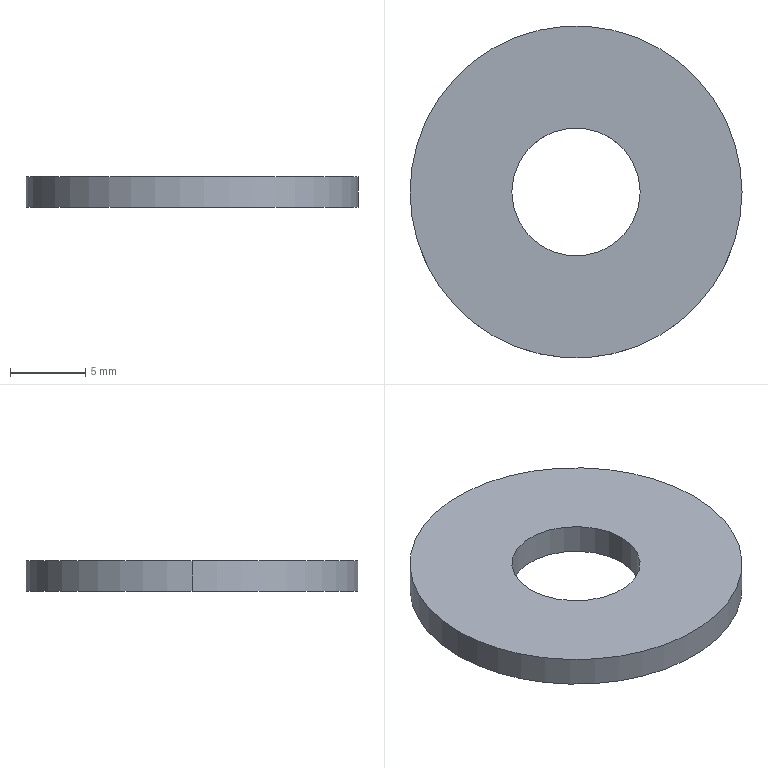Component | SolidWorks | 8mmLargeWasher-1 | 1 solid | 6 faces | box 22 x 22 x 2 mm | volume 647 mm3 | cylinder 4 | plane 2 | commonest cylinder face diameters 8.5 x2 22 x2
build123d program:
from build123d import *

# Parameters (mm, degrees)
SKETCH1_R           = 11
SKETCH1_R_2         = 4.25
BOSS_EXTRUDE1_DEPTH = 2


with BuildPart() as part:
    # Sketch1 → Boss-Extrude1 (new body)
    with BuildSketch(Plane.XY):
        with Locations((-70, -20)):
            Circle(SKETCH1_R)
        with Locations((-70, -20)):
            Circle(SKETCH1_R_2, mode=Mode.SUBTRACT)
    extrude(amount=BOSS_EXTRUDE1_DEPTH)


solid = part.part

# Placed as in the assembly
solid = solid.moved(Location((-426.612, -103.873, 2355.4), (0, 0, 0)))
STEP:
#1=COLOUR_RGB('',0.7922,0.8196,0.9333);
#2=FILL_AREA_STYLE_COLOUR('',#1);
#3=FILL_AREA_STYLE('',(#2));
#4=SURFACE_STYLE_FILL_AREA(#3);
#5=SURFACE_SIDE_STYLE('',(#4));
#6=SURFACE_STYLE_USAGE(.BOTH.,#5);
#7=PRESENTATION_STYLE_ASSIGNMENT((#6));
#8=CARTESIAN_POINT('',(-19.719,-4.877,92.732));
#9=VERTEX_POINT('',#8);
#10=CARTESIAN_POINT('',(-19.384,-4.877,92.732));
#11=VERTEX_POINT('',#10);
#12=CARTESIAN_POINT('',(-19.552,-4.877,92.732));
#13=DIRECTION('',(0.,0.,-1.));
#14=DIRECTION('',(1.,0.,0.));
#15=AXIS2_PLACEMENT_3D('',#12,#13,#14);
#16=CIRCLE('',#15,0.1673);
#17=EDGE_CURVE('',#9,#11,#16,.T.);
#18=ORIENTED_EDGE('',*,*,#17,.T.);
#19=CARTESIAN_POINT('',(-19.384,-4.877,92.811));
#20=VERTEX_POINT('',#19);
#21=CARTESIAN_POINT('',(-19.384,-4.877,92.732));
#22=DIRECTION('',(0.,-0.,1.));
#23=VECTOR('',#22,39.37);
#24=LINE('',#21,#23);
#25=EDGE_CURVE('',#11,#20,#24,.T.);
#26=ORIENTED_EDGE('',*,*,#25,.T.);
#27=CARTESIAN_POINT('',(-19.719,-4.877,92.811));
#28=VERTEX_POINT('',#27);
#29=CARTESIAN_POINT('',(-19.552,-4.877,92.811));
#30=DIRECTION('',(0.,0.,-1.));
#31=DIRECTION('',(1.,0.,0.));
#32=AXIS2_PLACEMENT_3D('',#29,#30,#31);
#33=CIRCLE('',#32,0.1673);
#34=EDGE_CURVE('',#28,#20,#33,.T.);
#35=ORIENTED_EDGE('',*,*,#34,.F.);
#36=CARTESIAN_POINT('',(-19.719,-4.877,92.732));
#37=DIRECTION('',(0.,-0.,1.));
#38=VECTOR('',#37,39.37);
#39=LINE('',#36,#38);
#40=EDGE_CURVE('',#9,#28,#39,.T.);
#41=ORIENTED_EDGE('',*,*,#40,.F.);
#42=EDGE_LOOP('',(#18,#26,#35,#41));
#43=FACE_OUTER_BOUND('',#42,.T.);
#44=CARTESIAN_POINT('',(-19.552,-4.877,92.732));
#45=DIRECTION('',(0.,-0.,1.));
#46=DIRECTION('',(-1.,0.,0.));
#47=AXIS2_PLACEMENT_3D('',#44,#45,#46);
#48=CYLINDRICAL_SURFACE('',#47,0.1673);
#49=ADVANCED_FACE('',(#43),#48,.F.);
#50=CARTESIAN_POINT('',(-19.119,-4.877,92.732));
#51=VERTEX_POINT('',#50);
#52=CARTESIAN_POINT('',(-19.985,-4.877,92.732));
#53=VERTEX_POINT('',#52);
#54=CARTESIAN_POINT('',(-19.552,-4.877,92.732));
#55=DIRECTION('',(0.,0.,-1.));
#56=DIRECTION('',(1.,0.,0.));
#57=AXIS2_PLACEMENT_3D('',#54,#55,#56);
#58=CIRCLE('',#57,0.4331);
#59=EDGE_CURVE('',#51,#53,#58,.T.);
#60=ORIENTED_EDGE('',*,*,#59,.F.);
#61=CARTESIAN_POINT('',(-19.119,-4.877,92.811));
#62=VERTEX_POINT('',#61);
#63=CARTESIAN_POINT('',(-19.119,-4.877,92.732));
#64=DIRECTION('',(0.,-0.,1.));
#65=VECTOR('',#64,39.37);
#66=LINE('',#63,#65);
#67=EDGE_CURVE('',#51,#62,#66,.T.);
#68=ORIENTED_EDGE('',*,*,#67,.T.);
#69=CARTESIAN_POINT('',(-19.985,-4.877,92.811));
#70=VERTEX_POINT('',#69);
#71=CARTESIAN_POINT('',(-19.552,-4.877,92.811));
#72=DIRECTION('',(0.,0.,-1.));
#73=DIRECTION('',(1.,0.,0.));
#74=AXIS2_PLACEMENT_3D('',#71,#72,#73);
#75=CIRCLE('',#74,0.4331);
#76=EDGE_CURVE('',#62,#70,#75,.T.);
#77=ORIENTED_EDGE('',*,*,#76,.T.);
#78=CARTESIAN_POINT('',(-19.985,-4.877,92.732));
#79=DIRECTION('',(0.,-0.,1.));
#80=VECTOR('',#79,39.37);
#81=LINE('',#78,#80);
#82=EDGE_CURVE('',#53,#70,#81,.T.);
#83=ORIENTED_EDGE('',*,*,#82,.F.);
#84=EDGE_LOOP('',(#60,#68,#77,#83));
#85=FACE_OUTER_BOUND('',#84,.T.);
#86=CARTESIAN_POINT('',(-19.552,-4.877,92.732));
#87=DIRECTION('',(0.,-0.,1.));
#88=DIRECTION('',(-1.,0.,0.));
#89=AXIS2_PLACEMENT_3D('',#86,#87,#88);
#90=CYLINDRICAL_SURFACE('',#89,0.4331);
#91=ADVANCED_FACE('',(#85),#90,.T.);
#92=CARTESIAN_POINT('',(-19.552,-4.877,92.732));
#93=DIRECTION('',(0.,0.,-1.));
#94=DIRECTION('',(1.,0.,0.));
#95=AXIS2_PLACEMENT_3D('',#92,#93,#94);
#96=CIRCLE('',#95,0.4331);
#97=EDGE_CURVE('',#53,#51,#96,.T.);
#98=ORIENTED_EDGE('',*,*,#97,.T.);
#99=ORIENTED_EDGE('',*,*,#59,.T.);
#100=EDGE_LOOP('',(#98,#99));
#101=FACE_OUTER_BOUND('',#100,.T.);
#102=ORIENTED_EDGE('',*,*,#17,.F.);
#103=CARTESIAN_POINT('',(-19.552,-4.877,92.732));
#104=DIRECTION('',(0.,0.,-1.));
#105=DIRECTION('',(1.,0.,0.));
#106=AXIS2_PLACEMENT_3D('',#103,#104,#105);
#107=CIRCLE('',#106,0.1673);
#108=EDGE_CURVE('',#11,#9,#107,.T.);
#109=ORIENTED_EDGE('',*,*,#108,.F.);
#110=EDGE_LOOP('',(#102,#109));
#111=FACE_BOUND('',#110,.T.);
#112=CARTESIAN_POINT('',(-19.552,-4.877,92.732));
#113=DIRECTION('',(0.,0.,-1.));
#114=DIRECTION('',(1.,-0.,0.));
#115=AXIS2_PLACEMENT_3D('',#112,#113,#114);
#116=PLANE('',#115);
#117=ADVANCED_FACE('',(#101,#111),#116,.T.);
#118=CARTESIAN_POINT('',(-19.552,-4.877,92.811));
#119=DIRECTION('',(0.,0.,-1.));
#120=DIRECTION('',(1.,0.,0.));
#121=AXIS2_PLACEMENT_3D('',#118,#119,#120);
#122=CIRCLE('',#121,0.4331);
#123=EDGE_CURVE('',#70,#62,#122,.T.);
#124=ORIENTED_EDGE('',*,*,#123,.F.);
#125=ORIENTED_EDGE('',*,*,#76,.F.);
#126=EDGE_LOOP('',(#124,#125));
#127=FACE_OUTER_BOUND('',#126,.T.);
#128=ORIENTED_EDGE('',*,*,#34,.T.);
#129=CARTESIAN_POINT('',(-19.552,-4.877,92.811));
#130=DIRECTION('',(0.,0.,-1.));
#131=DIRECTION('',(1.,0.,0.));
#132=AXIS2_PLACEMENT_3D('',#129,#130,#131);
#133=CIRCLE('',#132,0.1673);
#134=EDGE_CURVE('',#20,#28,#133,.T.);
#135=ORIENTED_EDGE('',*,*,#134,.T.);
#136=EDGE_LOOP('',(#128,#135));
#137=FACE_BOUND('',#136,.T.);
#138=CARTESIAN_POINT('',(-19.552,-4.877,92.811));
#139=DIRECTION('',(0.,0.,-1.));
#140=DIRECTION('',(1.,-0.,0.));
#141=AXIS2_PLACEMENT_3D('',#138,#139,#140);
#142=PLANE('',#141);
#143=ADVANCED_FACE('',(#127,#137),#142,.F.);
#144=ORIENTED_EDGE('',*,*,#67,.F.);
#145=ORIENTED_EDGE('',*,*,#97,.F.);
#146=ORIENTED_EDGE('',*,*,#82,.T.);
#147=ORIENTED_EDGE('',*,*,#123,.T.);
#148=EDGE_LOOP('',(#144,#145,#146,#147));
#149=FACE_OUTER_BOUND('',#148,.T.);
#150=CARTESIAN_POINT('',(-19.552,-4.877,92.732));
#151=DIRECTION('',(0.,-0.,1.));
#152=DIRECTION('',(-1.,0.,0.));
#153=AXIS2_PLACEMENT_3D('',#150,#151,#152);
#154=CYLINDRICAL_SURFACE('',#153,0.4331);
#155=ADVANCED_FACE('',(#149),#154,.T.);
#156=ORIENTED_EDGE('',*,*,#25,.F.);
#157=ORIENTED_EDGE('',*,*,#108,.T.);
#158=ORIENTED_EDGE('',*,*,#40,.T.);
#159=ORIENTED_EDGE('',*,*,#134,.F.);
#160=EDGE_LOOP('',(#156,#157,#158,#159));
#161=FACE_OUTER_BOUND('',#160,.T.);
#162=CARTESIAN_POINT('',(-19.552,-4.877,92.732));
#163=DIRECTION('',(0.,-0.,1.));
#164=DIRECTION('',(-1.,0.,0.));
#165=AXIS2_PLACEMENT_3D('',#162,#163,#164);
#166=CYLINDRICAL_SURFACE('',#165,0.1673);
#167=ADVANCED_FACE('',(#161),#166,.F.);
#168=CLOSED_SHELL('',(#49,#91,#117,#143,#155,#167));
#169=MANIFOLD_SOLID_BREP('',#168);
#170=STYLED_ITEM('',(#7),#169);
#171=PRESENTATION_LAYER_ASSIGNMENT('','',(#170));
#172=CARTESIAN_POINT('',(0.,0.,0.));
#173=DIRECTION('',(0.,0.,1.));
#174=DIRECTION('',(1.,0.,0.));
#175=AXIS2_PLACEMENT_3D('',#172,#173,#174);
#176=(LENGTH_UNIT()NAMED_UNIT(*)SI_UNIT($,.METRE.));
#177=LENGTH_MEASURE_WITH_UNIT(LENGTH_MEASURE(0.0254),#176);
#178=DIMENSIONAL_EXPONENTS(1.,0.,0.,0.,0.,0.,0.);
#179=(CONVERSION_BASED_UNIT('',#177)LENGTH_UNIT()NAMED_UNIT(#178));
#180=UNCERTAINTY_MEASURE_WITH_UNIT(LENGTH_MEASURE(0.00001),#179,'','');
#181=(NAMED_UNIT(*)PLANE_ANGLE_UNIT()SI_UNIT($,.RADIAN.));
#182=(NAMED_UNIT(*)SI_UNIT($,.STERADIAN.)SOLID_ANGLE_UNIT());
#183=(GEOMETRIC_REPRESENTATION_CONTEXT(3)GLOBAL_UNCERTAINTY_ASSIGNED_CONTEXT((#180))GLOBAL_UNIT_ASSIGNED_CONTEXT((#179,#181,#182))REPRESENTATION_CONTEXT('',''));
#184=ADVANCED_BREP_SHAPE_REPRESENTATION('',(#169,#175),#183);
#185=(LENGTH_UNIT()NAMED_UNIT(*)SI_UNIT($,.METRE.));
#186=LENGTH_MEASURE_WITH_UNIT(LENGTH_MEASURE(0.0254),#185);
#187=DIMENSIONAL_EXPONENTS(1.,0.,0.,0.,0.,0.,0.);
#188=(CONVERSION_BASED_UNIT('',#186)LENGTH_UNIT()NAMED_UNIT(#187));
#189=UNCERTAINTY_MEASURE_WITH_UNIT(LENGTH_MEASURE(0.00001),#188,'','');
#190=(NAMED_UNIT(*)PLANE_ANGLE_UNIT()SI_UNIT($,.RADIAN.));
#191=(NAMED_UNIT(*)SI_UNIT($,.STERADIAN.)SOLID_ANGLE_UNIT());
#192=(GEOMETRIC_REPRESENTATION_CONTEXT(3)GLOBAL_UNCERTAINTY_ASSIGNED_CONTEXT((#189))GLOBAL_UNIT_ASSIGNED_CONTEXT((#188,#190,#191))REPRESENTATION_CONTEXT('',''));
#193=MECHANICAL_DESIGN_GEOMETRIC_PRESENTATION_REPRESENTATION('',(#170),#192);